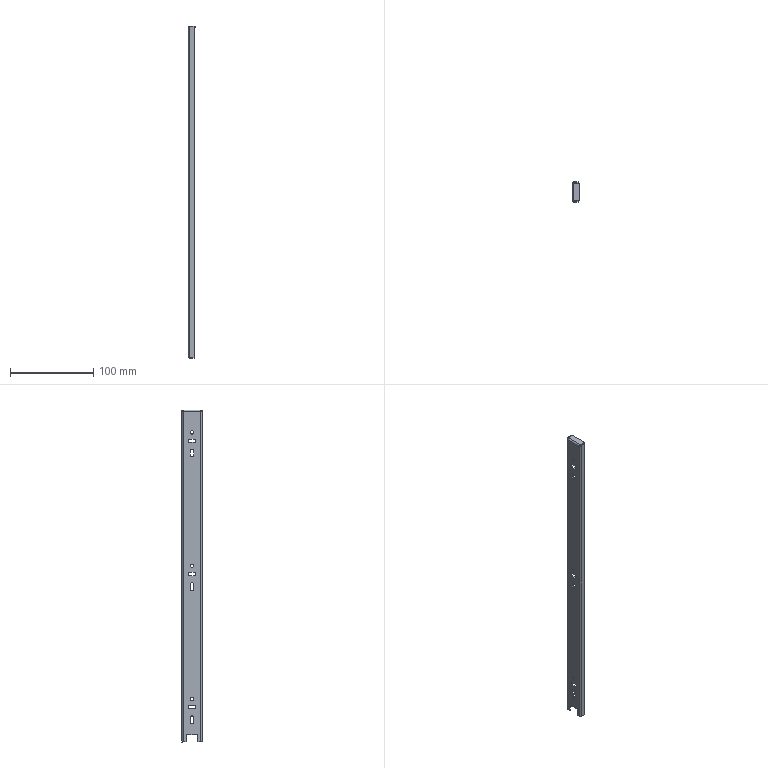Component | SolidWorks | PC-CAJ-P08-1_PC-CAJ-P16-1_Corredera C 400-1 | 1 solid | 66 faces | volume 16312 mm3 | plane 36 | cylinder 30 | commonest cylinder face diameters 4 x19 4.4 x5 1 x3 3.4 x3 | material Plain Carbon Steel